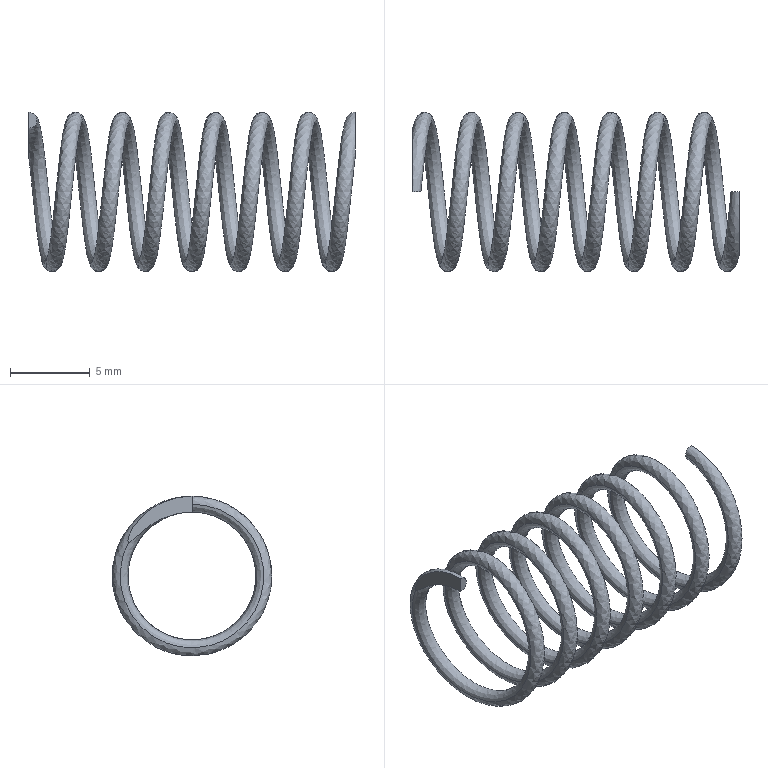Component | SolidWorks | LocatingSpring-1 | 1 solid | 6 faces | volume 154 mm3 | plane 4 | spline 2